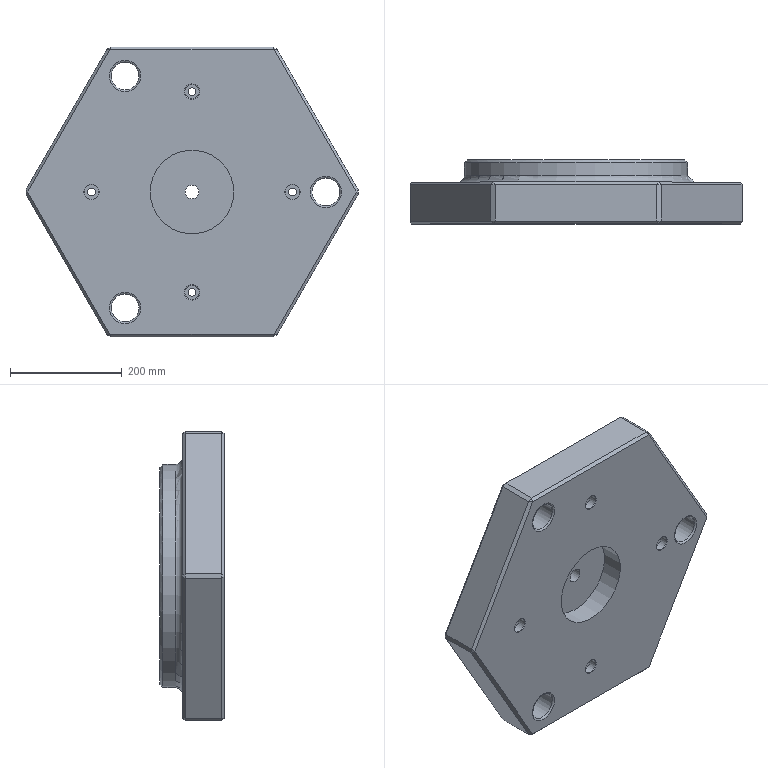Component | NX | BOTTOM_PLATE | 1 solid | 73 faces | volume 21252282 mm3 | plane 44 | cylinder 14 | torus 11 | spline 3 | cone 1 | commonest cylinder face diameters 14.2 x4 25.9 x4 50.2 x3 400 x1 25 x1 150 x1